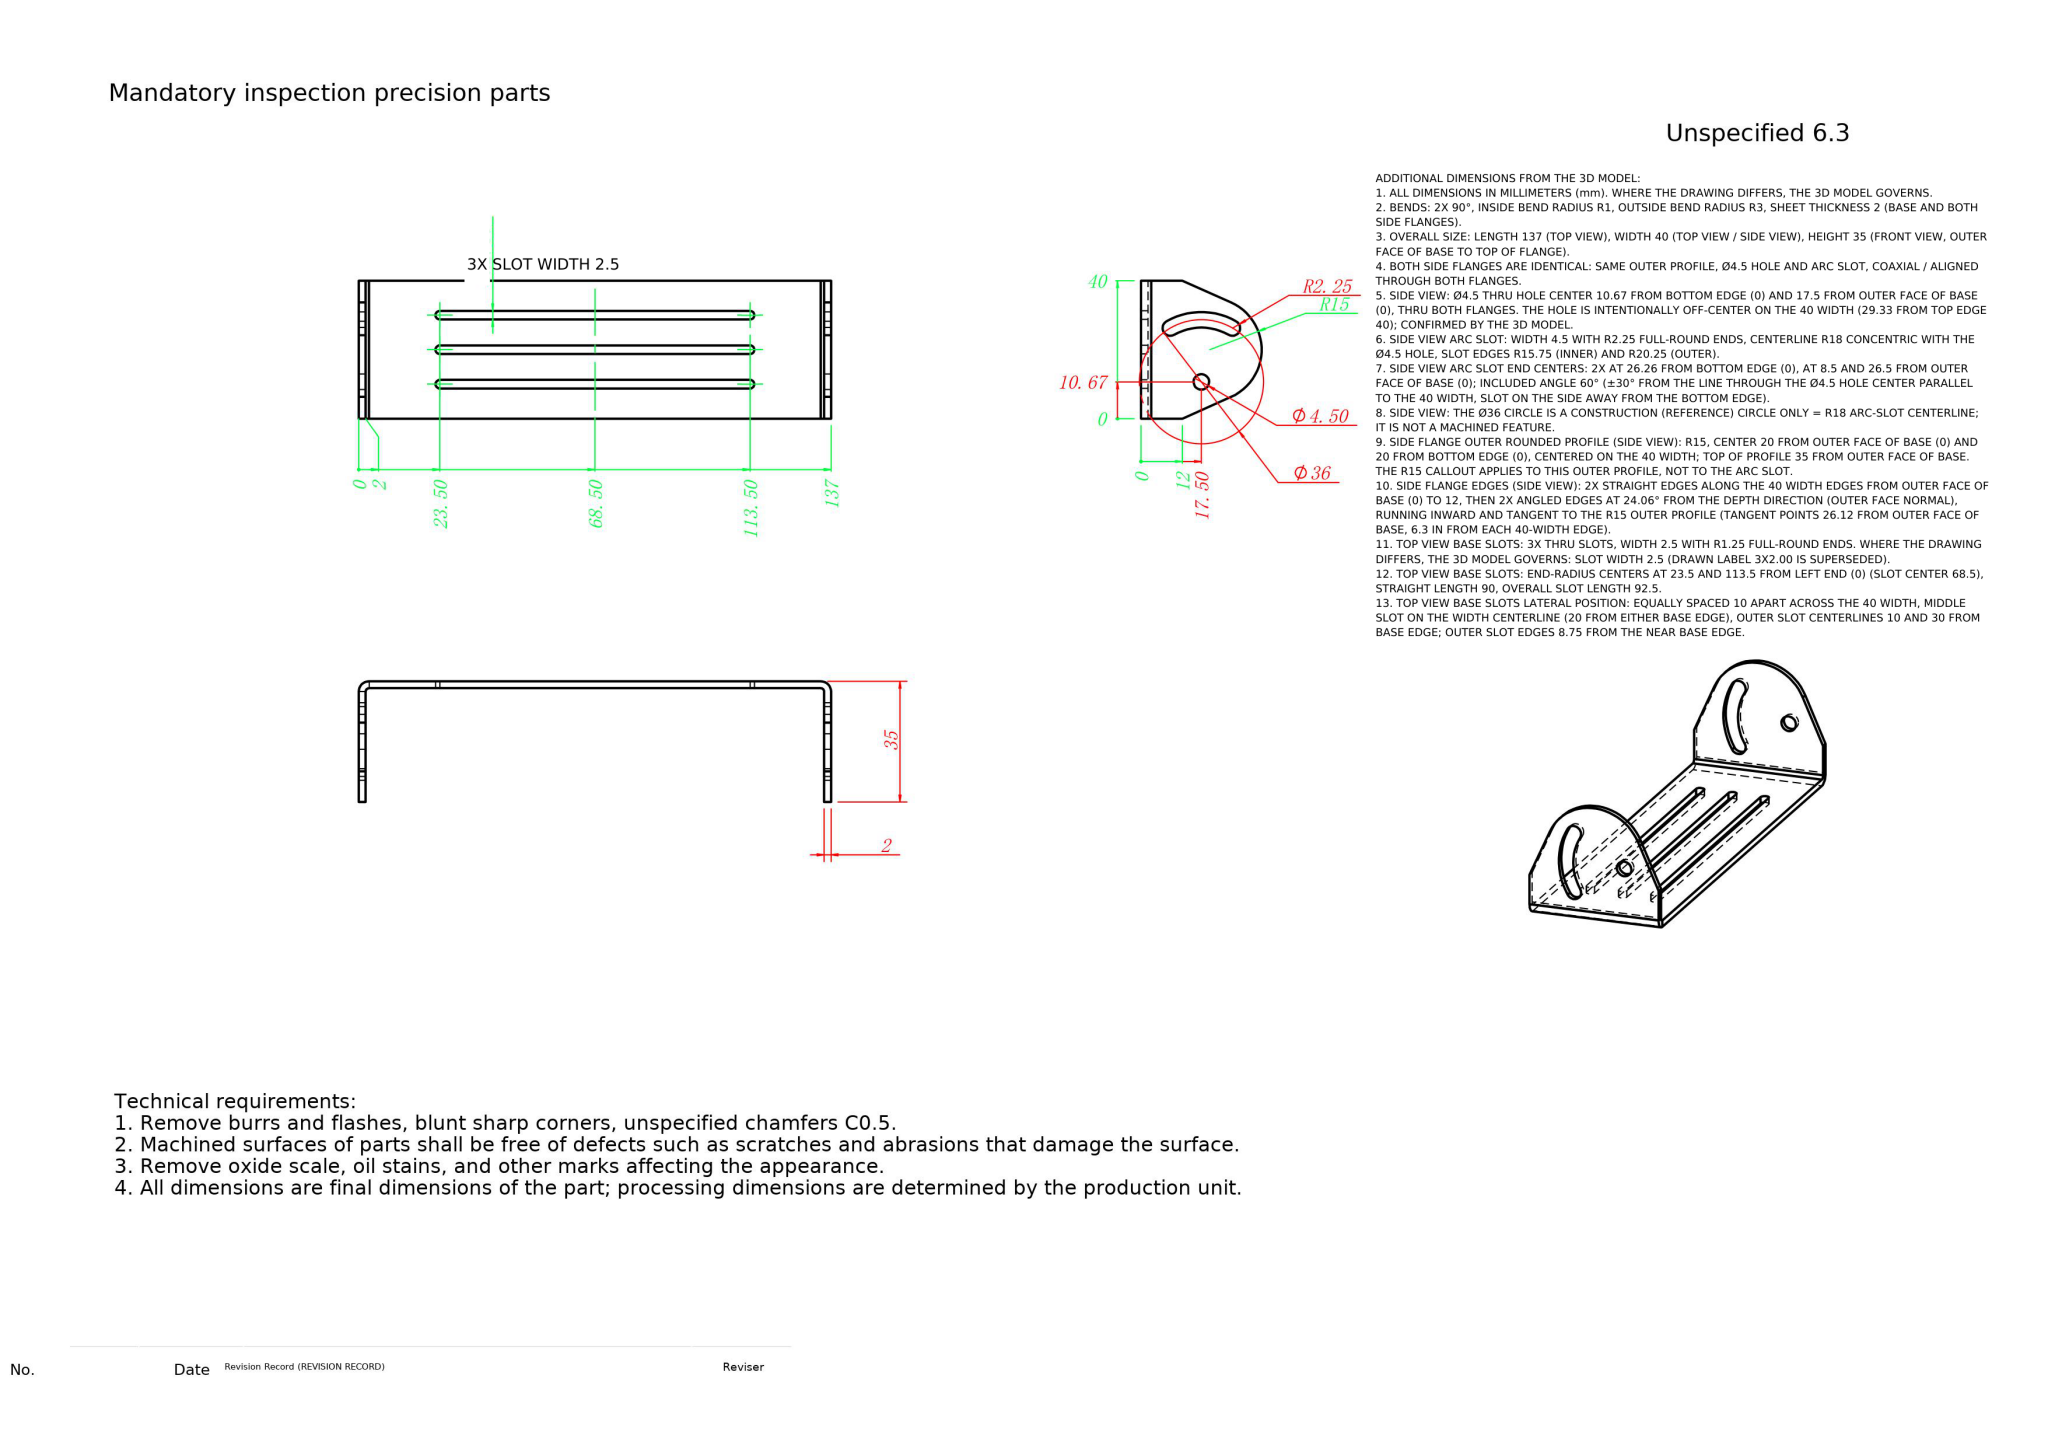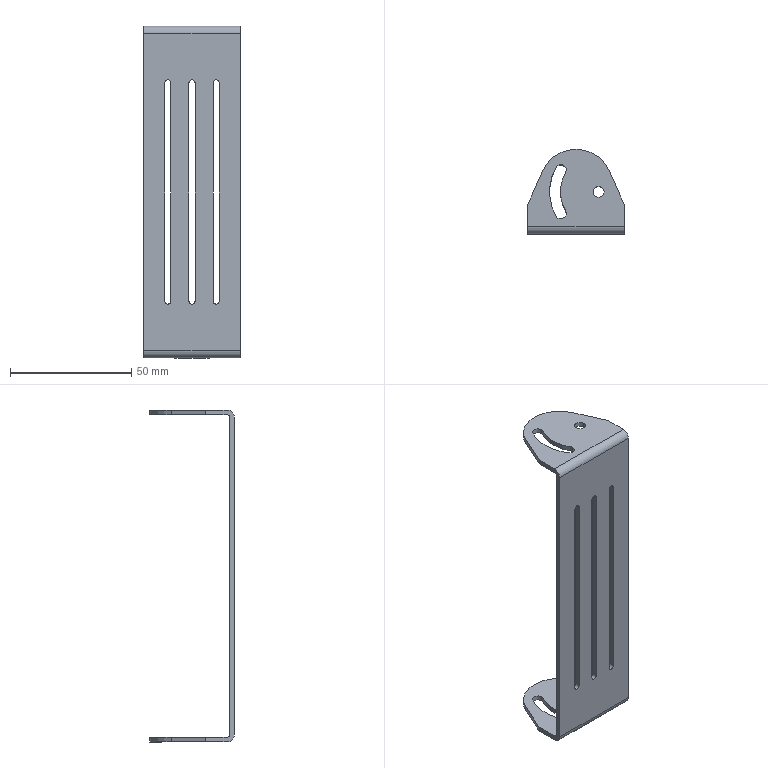Part | NX | mm | 1 solid | 52 faces | box 40 x 35 x 137 mm | volume 13180 mm3 | cylinder 32 | plane 20 | commonest cylinder face diameters 4.5 x12 2.5 x9 30 x3 6 x2 2 x2 40.5 x2 31.5 x2